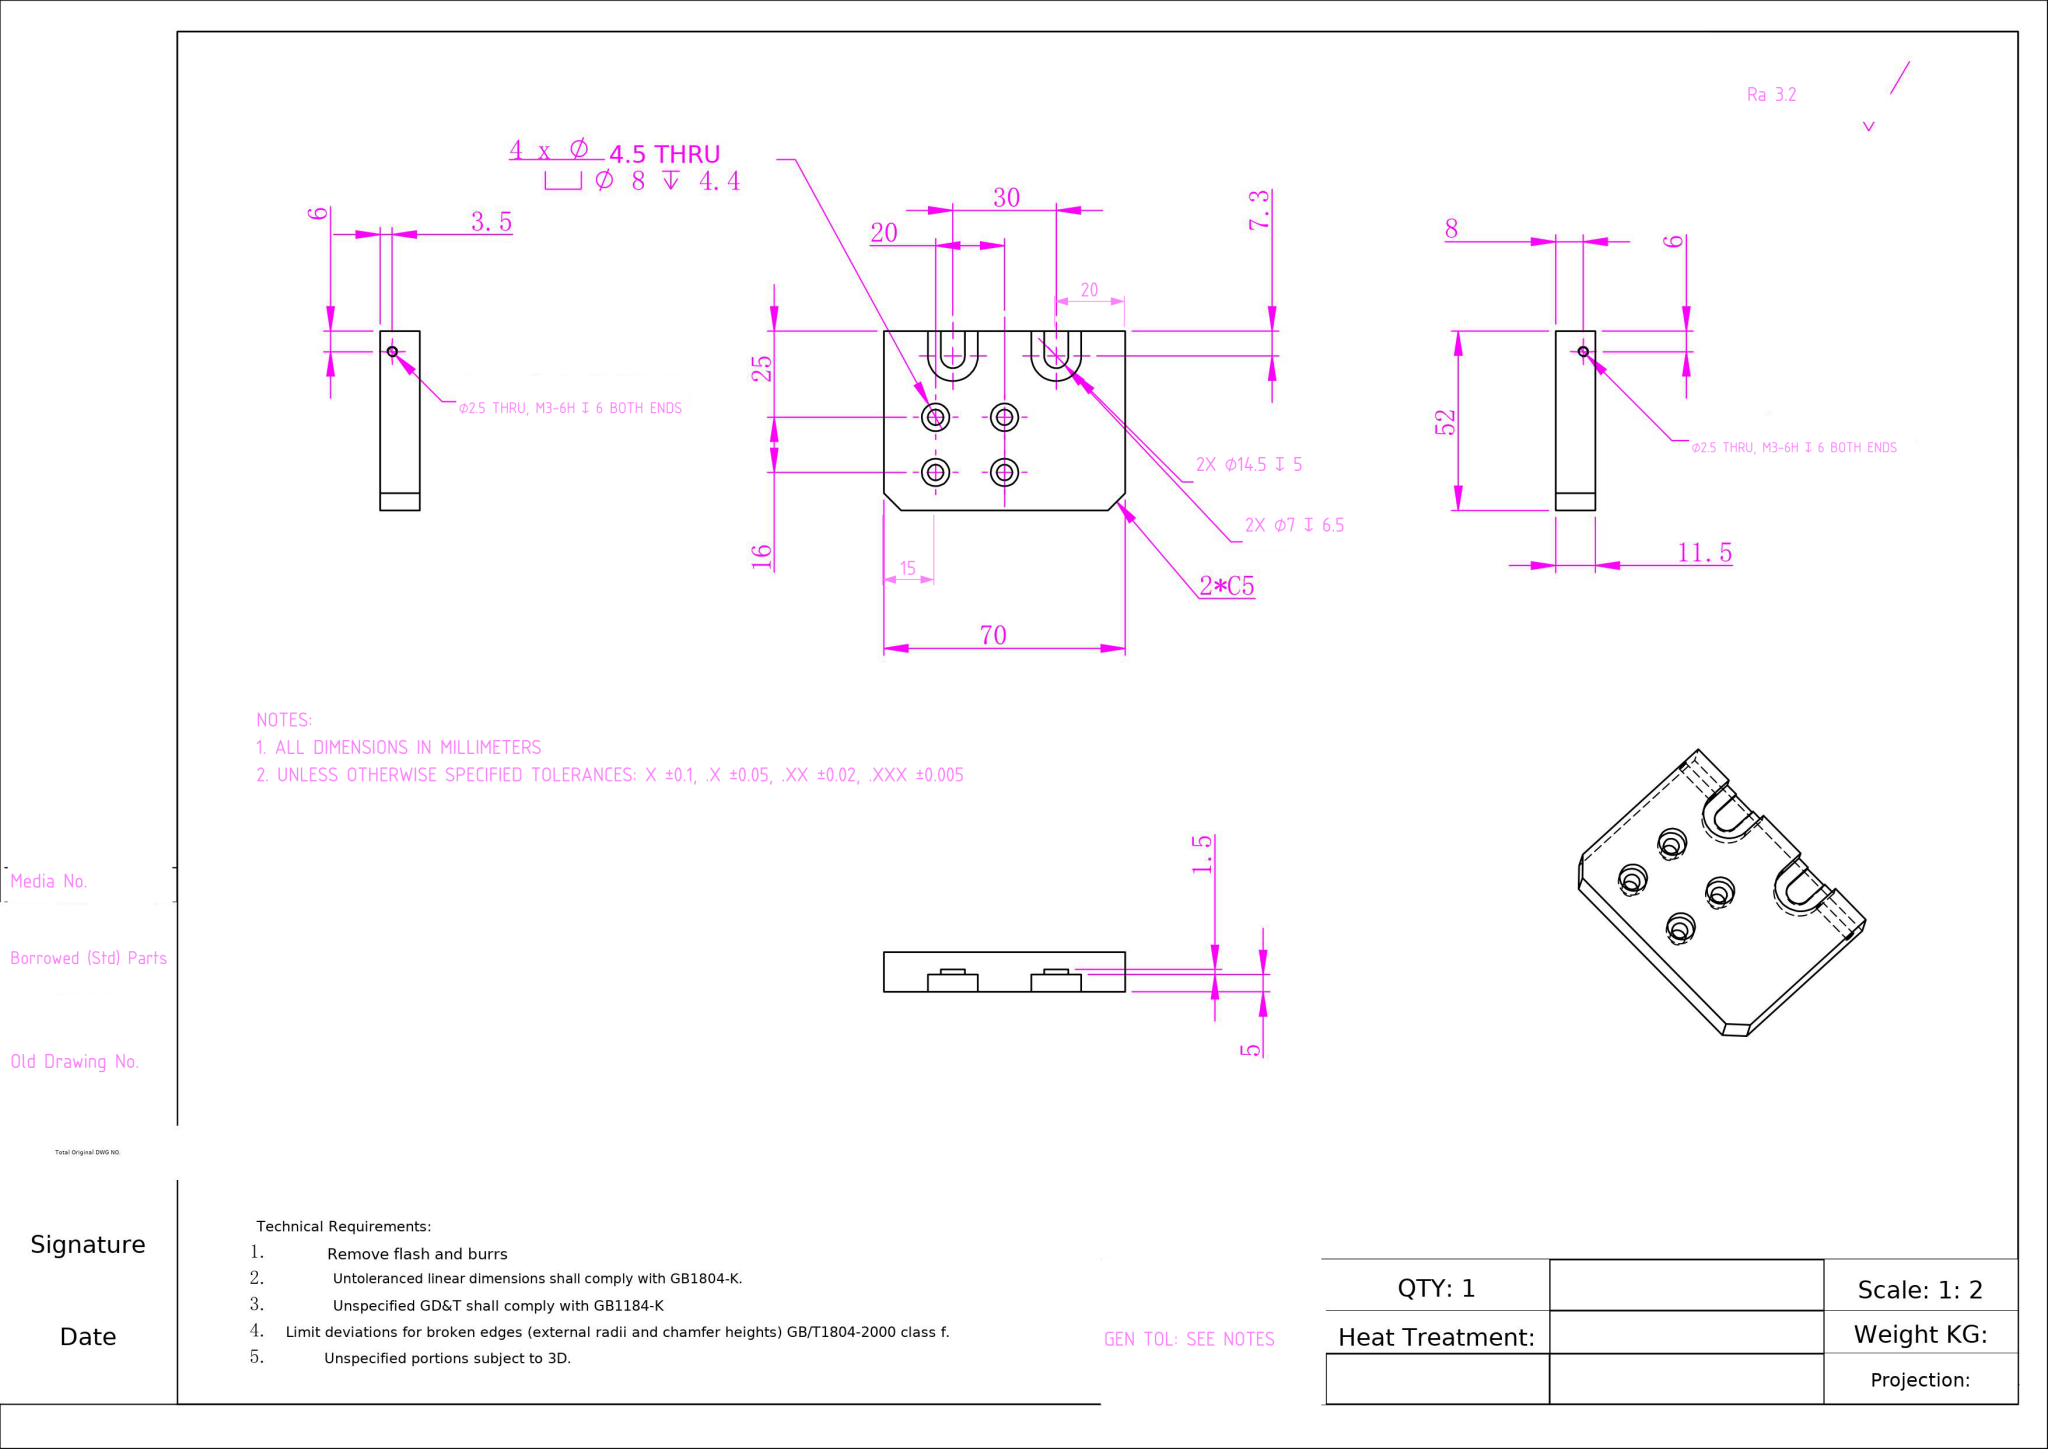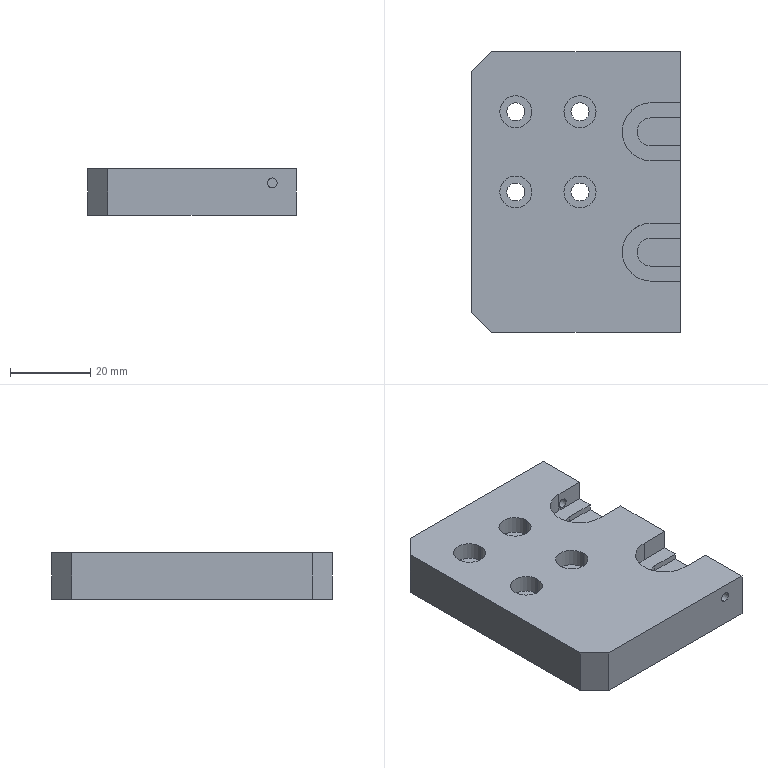Part | NX | mm | 1 solid | 48 faces | box 52 x 70 x 11.5 mm | volume 38024 mm3 | cylinder 24 | plane 24 | commonest cylinder face diameters 8 x8 4.5 x8 2.5 x4 14.5 x2 7 x2